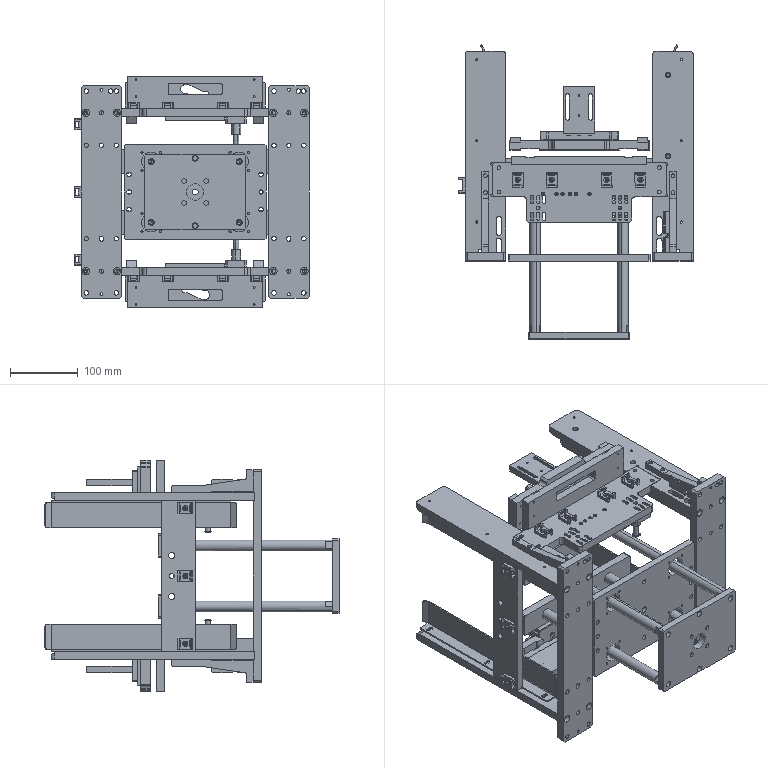Assembly | SolidWorks | mm | 65 component files | 65 solids | 2929 faces | box 346.2 x 434.2 x 342 mm | volume 3402690 mm3 | cylinder 1365 | plane 1260 | cone 216 | sphere 88 | commonest cylinder face diameters 0.6 x176 3.3 x164 4.5 x134 5.5 x96 6.6 x80 6 x79 4 x76 5 x66
Bill of materials:
01-1111 | 2 |  | Long, narrow, flat rectangular plate with small chamfered corners and an arrangement of round through holes laid out in rows, mostly three across, grouped near both ends and at about one-third and two-thirds of the length. Two small notches cut into one long edge.
02-1111 | 2 |  | Flat plate shaped like a T in plan. The wide main body has thinner, stepped-down tabs at each end, and each tab carries two round holes near its corners. A tab sticks out from one long edge, and near each of its ends sits a group of six parallel elongated slots arranged around a small central round hole.
03-1111 | 2 |  | Long rectangular bar with rounded corners at one end and a chamfered or angled edge at the same end. Near the other end it has a notched and stepped profile, a row of small holes, two elongated slots, and a hole in the end face. A long, shallow rectangular pocket or step is cut into one side edge in the middle of the bar, and there are a few widely spaced small holes on the top face.
04-1111 | 2 |  | Long rectangular bar very similar to unnamed part. It has the same stepped and notched end with an end-face hole, two slots and a small-hole cluster. It differs in having extra larger holes on the top face, a chamfer along the top edge at the far end, and a shallow step on the side edge where the other part has a long pocket.
05-1111 | 4 |  | Solid arm shaped roughly like an L. A tall rectangular block at one end has a horizontal round through hole. A tapered arm runs from the block, with its top surface sloping down to a level section near the far end. The level section has two vertical through holes, and there is a small step on the underside.
06-1111 | 4 |  | Long L-shaped angle that looks like bent sheet metal. It has an upright flange with rounded or chamfered end corners and a base flange with three elongated slots spaced along its length.
07-1111 | 1 |  | Rectangular bar or plate with four countersunk or conically shaped holes in one large face. Three round holes run along one narrow edge face, two larger and one smaller between them. There is a small step or rabbet along one long edge.
08-1111 | 2 |  | Thick, nearly square block with chamfered vertical corners. It has six round holes in two rows of three, with the middle hole of each row larger. A central hole has a larger counterbore or recess on the top face.
09-1111 | 4 |  | Small L-shaped bracket that looks like bent sheet metal. One flange has one long elongated slot. The other flange has two round holes near its outer corners. The outer corners are rounded.
10-1111 | 1 |  | Long, straight prismatic bar whose cross-section is a rectangle with one large angled chamfer, giving a five-sided profile. It has no holes or other features.
11-1111 | 2 |  | Stepped cylindrical pin. A slender shaft has a groove near its chamfered tip. The shaft joins a larger-diameter body that has one flat on its side. A short, reduced-diameter, chamfered spigot sits at the opposite end.
13-1111 | 2 |  | Thick rectangular plate with a rounded-rectangle through window in its upper middle. Five round holes run in a line near the bottom edge. Small holes sit near the end edges, shallow notches are cut into the top edge, and there is a step along one edge.
14-Z1-1111 | 2 |  | Elongated flat plate with a taller central section, an S-shaped curved through-slot, a 2x2 pattern of small holes on each end pad, and stepped thickness along the long edges.
17-1111 | 2 |  | Rectangular plate with two countersunk through-holes, chamfered top corners, and a stepped (L-shaped) cross-section.
18-1111 | 2 |  | Rectangular block with two long parallel through-slots and two small holes on the top face, three holes in one side face, and two lengthwise rectangular grooves on the underside.
19-1111 | 2 |  | I-shaped (dog-bone) bar: a narrow central web with three round through-holes, joining wider end pads that each have two elongated slots.
20-1111 | 4 |  | Thin flat rectangular plate with two elongated through-slots along its length and chamfered corners.
25-1111 | 4 |  | Rectangular bar with two round through-holes and a single angled bevel across one end.
21-1111 | 1 | S45C | Flat rectangular plate with four large circular openings, each surrounded by four small holes, plus medium holes on the centerline and along both short edges.
22-BF-1111 | 4 | 40CR | Long, slender cylindrical tube or rod with a central bore and a short, smaller-diameter step at one end.
23-1111 | 1 | A6061 | Flat rectangular plate with a large central through-bore, four small holes in a square around it, six perimeter holes, and chamfered corners.
24-1111 | 2 | A6061 | Flat rectangular bar with rounded corners and two counterbored through-holes near the ends.
RetainingRing~STWN8~MISUMI-1111 | 2 |  | Thin flat ring with a protruding tab that has an elongated slot; a split line passes radially through the tab and slot.
WireClip~M4-02~-1111 | 11 | PEEK | Rectangular block with a C/bracket-shaped profile: a solid base with a central round through-hole, and two raised end walls with inward lips forming rectangular through-passages.
Mates:
1. coincident | 01-1111-1 face at (-135.072, 406.224, 1393.056) dir (0, 1, 0) | 03-1111-1 face at (-135.072, 406.224, 1510.056) dir (0, -1, 0)
2. width | 01-1111-1 face at (-105.072, 408.224, 1236.056) dir (1, 0, 0) | 01-1111-1 face at (-165.072, 408.224, 1236.056) dir (-1, 0, 0) | 03-1111-1 face at (-165.072, 406.224, 1504.056) dir (-1, 0, 0) | 03-1111-1 face at (-105.072, 406.224, 1504.056) dir (1, 0, 0)
3. width | 03-1111-1 face at (-165.072, 406.224, 1516.056) dir (0, 0, 1) | 03-1111-1 face at (-165.072, 406.224, 1504.056) dir (0, 0, -1) | 01-1111-1 face at (-165.072, 406.224, 1516.056) dir (0, 0, -1) | 01-1111-1 face at (-165.072, 406.224, 1504.056) dir (0, 0, 1)
4. width | 04-1111-1 face at (-105.072, 406.224, 1270.056) dir (1, 0, 0) | 04-1111-1 face at (-165.072, 406.224, 1270.056) dir (-1, 0, 0) | 01-1111-1 face at (-105.072, 408.224, 1236.056) dir (1, 0, 0) | 01-1111-1 face at (-165.072, 408.224, 1236.056) dir (-1, 0, 0)
5. coincident | 01-1111-1 face at (-165.072, 408.224, 1550.056) dir (0, 0, 1) | 01-1111-2 face at (111.928, 408.224, 1550.056) dir (0, 0, 1)
6. coincident | 01-1111-1 face at (-135.072, 396.224, 1393.056) dir (0, -1, 0) | 01-1111-2 face at (141.928, 396.224, 1393.056) dir (0, -1, 0)
7. coincident | 01-1111-1 face at (-135.072, 408.224, 1393.056) dir (0, 1, 0) | 05-1111-1 face at (-140.072, 408.224, 1516.056) dir (0, -1, 0)
8. width | 01-1111-1 face at (-105.072, 408.224, 1236.056) dir (1, 0, 0) | 01-1111-1 face at (-165.072, 408.224, 1236.056) dir (-1, 0, 0) | 05-1111-1 face at (-140.072, 468.224, 1533.056) dir (-1, 0, 0) | 05-1111-1 face at (-130.072, 468.224, 1533.056) dir (1, 0, 0)
9. coincident | 01-1111-1 face at (-135.072, 408.224, 1393.056) dir (0, 1, 0) | 05-1111-3 face at (-130.072, 408.224, 1270.056) dir (0, -1, 0)
10. width | 01-1111-1 face at (-105.072, 408.224, 1236.056) dir (1, 0, 0) | 01-1111-1 face at (-165.072, 408.224, 1236.056) dir (-1, 0, 0) | 05-1111-3 face at (-140.072, 468.224, 1253.056) dir (-1, 0, 0) | 05-1111-3 face at (-130.072, 468.224, 1253.056) dir (1, 0, 0)
11. coincident | 03-1111-1 face at (-165.072, 406.224, 1516.056) dir (0, 0, 1) | 05-1111-1 face at (-140.072, 528.224, 1516.056) dir (0, 0, -1)
12. width | 03-1111-1 face at (-165.072, 406.224, 1516.056) dir (0, 0, 1) | 04-1111-1 face at (-165.072, 406.224, 1270.056) dir (0, 0, -1) | 07-1111-1 face at (-153.072, 543.224, 1282.056) dir (0, 0, -1) | 07-1111-1 face at (-153.072, 543.224, 1504.056) dir (0, 0, 1)
13. coincident | 04-1111-1 face at (-135.072, 706.224, 1276.056) dir (0, 0, -1) | 02-1111-3 face at (3.428, 516.224, 1276.056) dir (0, 0, 1)
14. width | 04-1111-1 face at (-105.072, 541.224, 1276.056) dir (0, -1, 0) | 04-1111-1 face at (-105.072, 491.224, 1276.056) dir (0, 1, 0) | 02-1111-3 face at (131.928, 491.224, 1282.056) dir (0, -1, 0) | 02-1111-3 face at (131.928, 541.224, 1282.056) dir (0, 1, 0)
15. coincident | 04-1111-1 face at (-105.072, 406.224, 1270.056) dir (1, 0, 0) | 02-1111-3 face at (-105.072, 491.224, 1276.056) dir (-1, 0, 0)
16. coincident | 04-1111-1 face at (-165.072, 406.224, 1270.056) dir (0, 0, -1) | 05-1111-3 face at (-130.072, 528.224, 1270.056) dir (0, 0, 1)
17. coincident | 04-1111-1 face at (-165.072, 406.224, 1282.056) dir (0, 0, 1) | 06-1111-6 face at (-135.572, 441.224, 1282.056) dir (0, 0, -1)
18. coincident | 04-1111-1 face at (-135.072, 706.224, 1276.056) dir (0, 1, 0) | 06-1111-6 face at (-138.308, 706.224, 1284.792) dir (0, 1, 0)
19. distance | 06-1111-6 face at (-135.572, 441.224, 1322.056) dir (1, 0, 0) | 04-1111-1 face at (-105.072, 406.224, 1270.056) dir (1, 0, 0)
20. width | 04-1111-2 face at (171.928, 406.224, 1516.056) dir (0, 0, 1) | 04-1111-2 face at (171.928, 406.224, 1504.056) dir (0, 0, -1) | 01-1111-2 face at (111.928, 406.224, 1504.056) dir (0, 0, 1) | 01-1111-2 face at (111.928, 406.224, 1516.056) dir (0, 0, -1)
21. width | 04-1111-2 face at (171.928, 406.224, 1516.056) dir (1, 0, 0) | 04-1111-2 face at (111.928, 406.224, 1516.056) dir (-1, 0, 0) | 01-1111-2 face at (171.928, 408.224, 1236.056) dir (1, 0, 0) | 01-1111-2 face at (111.928, 408.224, 1236.056) dir (-1, 0, 0)
22. width | 01-1111-2 face at (111.928, 406.224, 1282.056) dir (0, 0, -1) | 01-1111-2 face at (111.928, 406.224, 1270.056) dir (0, 0, 1) | 03-1111-2 face at (171.928, 406.224, 1270.056) dir (0, 0, -1) | 03-1111-2 face at (171.928, 406.224, 1282.056) dir (0, 0, 1)
23. width | 03-1111-2 face at (111.928, 406.224, 1282.056) dir (-1, 0, 0) | 03-1111-2 face at (171.928, 406.224, 1282.056) dir (1, 0, 0) | 01-1111-2 face at (171.928, 408.224, 1236.056) dir (1, 0, 0) | 01-1111-2 face at (111.928, 408.224, 1236.056) dir (-1, 0, 0)
24. coincident | 01-1111-2 face at (141.928, 408.224, 1393.056) dir (0, 1, 0) | 05-1111-2 face at (136.928, 408.224, 1516.056) dir (0, -1, 0)
25. width | 01-1111-2 face at (111.928, 408.224, 1236.056) dir (-1, 0, 0) | 01-1111-2 face at (171.928, 408.224, 1236.056) dir (1, 0, 0) | 05-1111-2 face at (136.928, 468.224, 1533.056) dir (-1, 0, 0) | 05-1111-2 face at (146.928, 468.224, 1533.056) dir (1, 0, 0)
26. coincident | 01-1111-2 face at (141.928, 408.224, 1393.056) dir (0, 1, 0) | 05-1111-4 face at (146.928, 408.224, 1270.056) dir (0, -1, 0)
27. width | 01-1111-2 face at (111.928, 408.224, 1236.056) dir (-1, 0, 0) | 01-1111-2 face at (171.928, 408.224, 1236.056) dir (1, 0, 0) | 05-1111-4 face at (146.928, 468.224, 1253.056) dir (1, 0, 0) | 05-1111-4 face at (136.928, 468.224, 1253.056) dir (-1, 0, 0)
28. coincident | 03-1111-2 face at (171.928, 406.224, 1270.056) dir (0, 0, -1) | 05-1111-4 face at (146.928, 528.224, 1270.056) dir (0, 0, 1)
29. coincident | 04-1111-2 face at (171.928, 406.224, 1516.056) dir (0, 0, 1) | 05-1111-2 face at (136.928, 528.224, 1516.056) dir (0, 0, -1)
30. coincident | 04-1111-2 face at (171.928, 406.224, 1504.056) dir (0, 0, -1) | 06-1111-5 face at (142.428, 441.224, 1504.056) dir (0, 0, 1)
31. coincident | 04-1111-2 face at (141.928, 706.224, 1510.056) dir (0, 1, 0) | 06-1111-5 face at (145.165, 706.224, 1501.319) dir (0, 1, 0)
32. distance | 06-1111-5 face at (142.428, 441.224, 1464.056) dir (-1, 0, 0) | 04-1111-2 face at (111.928, 406.224, 1516.056) dir (-1, 0, 0)
33. coincident | 04-1111-1 face at (-165.072, 406.224, 1270.056) dir (-1, 0, 0) | 07-1111-1 face at (-165.072, 518.224, 1393.056) dir (-1, 0, 0)
34. coincident | 04-1111-2 face at (171.928, 406.224, 1516.056) dir (0, 0, 1) | 09-1111-1 face at (147.928, 399.224, 1516.056) dir (0, 0, -1)
35. parallel | 04-1111-2 face at (141.928, 706.224, 1510.056) dir (0, 1, 0) | 09-1111-1 face at (129.928, 431.224, 1518.792) dir (0, 1, 0)
36. distance | 09-1111-1 face at (147.928, 399.224, 1518.056) dir (1, 0, 0) | 04-1111-2 face at (171.928, 406.224, 1516.056) dir (1, 0, 0)
37. distance | 09-1111-1 face at (129.928, 431.224, 1518.792) dir (0, 1, 0) | 04-1111-2 face at (141.928, 706.224, 1510.056) dir (0, 1, 0)
38. coincident | 09-1111-1 face at (129.928, 431.224, 1518.792) dir (0, 1, 0) | 09-1111-12 face at (130.665, 431.224, 1267.319) dir (0, 1, 0)
39. coincident | 09-1111-1 face at (127.928, 399.224, 1516.056) dir (-1, 0, 0) | 09-1111-12 face at (127.928, 431.224, 1270.056) dir (-1, 0, 0)
40. coincident | 03-1111-2 face at (171.928, 406.224, 1270.056) dir (0, 0, -1) | 09-1111-12 face at (147.928, 431.224, 1270.056) dir (0, 0, 1)
41. coincident | 04-1111-1 face at (-165.072, 406.224, 1282.056) dir (0, 0, 1) | 10-1111-1 face at (-135.572, 406.224, 1282.056) dir (0, 0, -1)
42. coincident | 06-1111-6 face at (-135.572, 441.224, 1322.056) dir (1, 0, 0) | 10-1111-1 face at (-135.572, 406.224, 1282.056) dir (-1, 0, 0)
43. distance | 10-1111-1 face at (-128.072, 696.224, 1291.056) dir (0, 1, 0) | 04-1111-1 face at (-135.072, 706.224, 1276.056) dir (0, 1, 0)
44. distance | 07-1111-1 face at (-153.072, 543.224, 1282.056) dir (0, 1, 0) | 01-1111-1 face at (-135.072, 408.224, 1393.056) dir (0, 1, 0)
45. coincident | 11-1111-1 face at (63.928, 474.724, 1327.156) dir (0, 0, 1) | RetainingRing~STWN8~MISUMI-1111-1 face at (70.259, 473.944, 1327.156) dir (0, 0, -1)
46. concentric | 11-1111-1 face at (63.928, 474.724, 1290.056) dir (0, 0, -1) r 4 | RetainingRing~STWN8~MISUMI-1111-1 face at (63.928, 474.724, 1327.956) dir (0, 0, 1) r 3.8
47. coincident | 03-1111-1 face at (-135.072, 706.224, 1510.056) dir (0, 0, 1) | 02-1111-4 face at (3.428, 516.224, 1510.056) dir (0, 0, -1)
48. width | 02-1111-4 face at (-125.072, 541.224, 1504.056) dir (0, 1, 0) | 02-1111-4 face at (-125.072, 491.224, 1504.056) dir (0, -1, 0) | 03-1111-1 face at (-105.072, 541.224, 1510.056) dir (0, -1, 0) | 03-1111-1 face at (-105.072, 491.224, 1510.056) dir (0, 1, 0)
49. coincident | 03-1111-1 face at (-125.072, 541.224, 1510.056) dir (1, 0, 0) | 02-1111-4 face at (-125.072, 541.224, 1504.056) dir (-1, 0, 0)
50. coincident | 04-1111-2 face at (131.928, 541.224, 1510.056) dir (-1, 0, 0) | 02-1111-4 face at (131.928, 541.224, 1504.056) dir (1, 0, 0)
51. profile center | 11-1111-1 face at (64.268, 479.713, 1290.056) dir (0, 0, -1) | 08-1111-2 face at (63.928, 474.724, 1290.056) dir (0, 0, 1)
52. profile center | 11-1111-2 face at (60.777, 478.607, 1496.056) dir (0, 0, 1) | 08-1111-3 face at (63.928, 474.724, 1496.056) dir (0, 0, -1)
53. concentric | 11-1111-2 face at (63.928, 474.724, 1496.056) dir (0, 0, 1) r 4 | RetainingRing~STWN8~MISUMI-1111-2 face at (63.928, 474.724, 1458.956) dir (0, 0, 1) r 3.8
54. coincident | 11-1111-2 face at (63.928, 474.724, 1458.956) dir (0, 0, -1) | RetainingRing~STWN8~MISUMI-1111-2 face at (70.258, 473.937, 1458.956) dir (0, 0, 1)
55. coincident | 02-1111-4 face at (3.428, 516.224, 1504.056) dir (0, 0, -1) | 08-1111-3 face at (63.928, 474.724, 1504.056) dir (0, 0, 1)
56. concentric | 02-1111-4 face at (63.928, 474.724, 1504.056) dir (0, 0, 1) r 2.75 | 08-1111-3 face at (63.928, 474.724, 1504.056) dir (0, 0, 1) r 5
57. parallel | 02-1111-4 face at (80.928, 453.224, 1516.056) dir (1, 0, 0) | 08-1111-3 face at (78.928, 492.224, 1504.056) dir (1, 0, 0)
58. concentric | 02-1111-3 face at (63.928, 474.724, 1282.056) dir (0, 0, -1) r 2.75 | 08-1111-2 face at (63.928, 474.724, 1282.056) dir (0, 0, -1) r 5
59. coincident | 02-1111-3 face at (3.428, 516.224, 1282.056) dir (0, 0, 1) | 08-1111-2 face at (63.928, 474.724, 1282.056) dir (0, 0, -1)
60. parallel | 02-1111-3 face at (80.928, 453.224, 1270.056) dir (1, 0, 0) | 08-1111-2 face at (78.928, 492.224, 1282.056) dir (1, 0, 0)
61. coincident | 03-1111-2 face at (171.928, 406.224, 1282.056) dir (0, 0, 1) | 06-1111-3 face at (142.428, 706.224, 1282.056) dir (0, 0, -1)
62. distance | 06-1111-3 face at (142.428, 706.224, 1322.056) dir (-1, 0, 0) | 03-1111-2 face at (111.928, 406.224, 1282.056) dir (-1, 0, 0)
63. coincident | 03-1111-2 face at (141.928, 706.224, 1276.056) dir (0, 1, 0) | 06-1111-3 face at (144.428, 706.224, 1284.792) dir (0, 1, 0)
64. coincident | 03-1111-1 face at (-165.072, 406.224, 1504.056) dir (0, 0, -1) | 06-1111-4 face at (-135.572, 706.224, 1504.056) dir (0, 0, 1)
65. distance | 06-1111-4 face at (-135.572, 706.224, 1464.056) dir (1, 0, 0) | 03-1111-1 face at (-105.072, 406.224, 1504.056) dir (1, 0, 0)
66. coincident | 03-1111-1 face at (-135.072, 706.224, 1510.056) dir (0, 1, 0) | 06-1111-4 face at (-137.572, 706.224, 1501.319) dir (0, 1, 0)
67. coincident | 02-1111-3 face at (3.428, 516.224, 1270.056) dir (0, 0, -1) | 12-DividingMechanism-1111-2/13-1111-1 face at (103.428, 541.224, 1270.056) dir (0, 0, 1)
68. coincident | 02-1111-3 face at (131.928, 541.224, 1282.056) dir (0, 1, 0) | 12-DividingMechanism-1111-2/13-1111-1 face at (3.428, 541.224, 1252.056) dir (0, -1, 0)
69. coincident | 02-1111-4 face at (-125.072, 541.224, 1504.056) dir (0, 1, 0) | 12-DividingMechanism-1111-1/13-1111-1 face at (3.428, 541.224, 1534.056) dir (0, -1, 0)
70. coincident | 02-1111-4 face at (3.428, 516.224, 1516.056) dir (0, 0, 1) | 12-DividingMechanism-1111-1/13-1111-1 face at (-96.572, 541.224, 1516.056) dir (0, 0, -1)
71. coincident | 01-1111-1 face at (-135.072, 396.224, 1393.056) dir (0, -1, 0) | 20-MaterialTrayLifting-1111-1/21-1111-1 face at (3.428, 396.224, 1393.056) dir (0, -1, 0)
72. width | 01-1111-1 face at (-165.072, 408.224, 1236.056) dir (0, 0, -1) | 01-1111-1 face at (-165.072, 408.224, 1550.056) dir (0, 0, 1) | 20-MaterialTrayLifting-1111-1/21-1111-1 face at (-101.572, 406.224, 1323.056) dir (0, 0, -1) | 20-MaterialTrayLifting-1111-1/21-1111-1 face at (-101.572, 406.224, 1463.056) dir (0, 0, 1)
73. width | 01-1111-1 face at (-105.072, 408.224, 1236.056) dir (1, 0, 0) | 01-1111-2 face at (111.928, 408.224, 1236.056) dir (-1, 0, 0) | 20-MaterialTrayLifting-1111-1/21-1111-1 face at (-101.572, 406.224, 1323.056) dir (-1, 0, 0) | 20-MaterialTrayLifting-1111-1/21-1111-1 face at (108.428, 406.224, 1323.056) dir (1, 0, 0)
74. concentric | 02-1111-4 face at (93.928, 516.224, 1516.056) dir (0, 0, 1) r 1.65 | WireClip~M4-02~-1111-3 face at (93.928, 516.224, 1520.356) dir (0, 0, 1) r 2.25
75. coincident | WireClip~M4-02~-1111-5 face at (-45.005, 507.861, 1520.356) dir (0, 0, 1) | WireClip~M4-02~-1111-6 face at (-95.005, 507.861, 1520.356) dir (0, 0, 1)
76. coincident | WireClip~M4-02~-1111-4 face at (35.995, 507.861, 1520.356) dir (0, 0, 1) | WireClip~M4-02~-1111-5 face at (-45.005, 507.861, 1520.356) dir (0, 0, 1)
77. coincident | WireClip~M4-02~-1111-3 face at (85.995, 507.861, 1520.356) dir (0, 0, 1) | WireClip~M4-02~-1111-4 face at (35.995, 507.861, 1520.356) dir (0, 0, 1)
78. concentric | 02-1111-4 face at (43.928, 516.224, 1516.056) dir (0, 0, 1) r 1.65 | WireClip~M4-02~-1111-4 face at (43.928, 516.224, 1520.356) dir (0, 0, 1) r 4
79. concentric | 02-1111-4 face at (-37.072, 516.224, 1516.056) dir (0, 0, 1) r 1.65 | WireClip~M4-02~-1111-5 face at (-37.072, 516.224, 1520.356) dir (0, 0, 1) r 4
80. concentric | 02-1111-4 face at (-87.072, 516.224, 1516.056) dir (0, 0, 1) r 1.65 | WireClip~M4-02~-1111-6 face at (-87.072, 516.224, 1520.356) dir (0, 0, 1) r 4
81. coincident | 07-1111-1 face at (-165.072, 518.224, 1393.056) dir (-1, 0, 0) | WireClip~M4-02~-1111-11 face at (-165.072, 496.988, 1401.145) dir (1, 0, 0)
82. concentric | 07-1111-1 face at (-165.072, 508.224, 1393.056) dir (-1, 0, 0) r 1.65 | WireClip~M4-02~-1111-11 face at (-169.372, 508.224, 1393.056) dir (-1, 0, 0) r 4
83. coincident | WireClip~M4-02~-1111-14 face at (-169.372, 499.861, 1285.122) dir (-1, 0, 0) | WireClip~M4-02~-1111-15 face at (-169.372, 499.861, 1485.122) dir (-1, 0, 0)
84. coincident | WireClip~M4-02~-1111-11 face at (-169.372, 499.861, 1385.122) dir (-1, 0, 0) | WireClip~M4-02~-1111-14 face at (-169.372, 499.861, 1285.122) dir (-1, 0, 0)
85. concentric | 07-1111-1 face at (-165.072, 508.224, 1493.056) dir (-1, 0, 0) r 1.65 | WireClip~M4-02~-1111-15 face at (-169.372, 508.224, 1493.056) dir (-1, 0, 0) r 4
86. concentric | 07-1111-1 face at (-165.072, 508.224, 1293.056) dir (-1, 0, 0) r 1.65 | WireClip~M4-02~-1111-14 face at (-169.372, 508.224, 1293.056) dir (-1, 0, 0) r 4
87. coincident | 04-1111-1 face at (-165.072, 406.224, 1282.056) dir (0, 0, 1) | 07-1111-1 face at (-153.072, 543.224, 1282.056) dir (0, 0, -1)
88. width | 01-1111-1 face at (-165.072, 408.224, 1236.056) dir (0, 0, -1) | 01-1111-1 face at (-165.072, 408.224, 1550.056) dir (0, 0, 1) | 04-1111-1 face at (-165.072, 406.224, 1270.056) dir (0, 0, -1) | 03-1111-1 face at (-165.072, 406.224, 1516.056) dir (0, 0, 1)
89. coincident | 03-1111-1 face at (-165.072, 406.224, 1516.056) dir (0, 0, 1) | 04-1111-2 face at (171.928, 406.224, 1516.056) dir (0, 0, 1)
90. coincident | 03-1111-2 face at (171.928, 406.224, 1270.056) dir (0, 0, -1) | 04-1111-1 face at (-165.072, 406.224, 1270.056) dir (0, 0, -1)
91. coincident | 01-1111-1 face at (-135.072, 396.224, 1393.056) dir (0, -1, 0) | 01-1111-2 face at (141.928, 396.224, 1393.056) dir (0, -1, 0)
92. width | 03-1111-2 face at (111.928, 406.224, 1282.056) dir (-1, 0, 0) | 04-1111-1 face at (-105.072, 406.224, 1270.056) dir (1, 0, 0) | 12-DividingMechanism-1111-2/14-Z1-1111-1 face at (106.678, 573.824, 1222.056) dir (1, 0, 0) | 12-DividingMechanism-1111-2/14-Z1-1111-1 face at (-99.822, 573.824, 1222.056) dir (-1, 0, 0)
93. coincident | 12-DividingMechanism-1111-1/14-Z1-1111-1 face at (-99.822, 573.824, 1564.056) dir (-1, 0, 0) | 12-DividingMechanism-1111-2/14-Z1-1111-1 face at (-99.822, 573.824, 1222.056) dir (-1, 0, 0)
94. coincident | 01-1111-1 face at (-135.072, 406.224, 1393.056) dir (0, 1, 0) | 04-1111-1 face at (-135.072, 406.224, 1276.056) dir (0, -1, 0)
95. coincident | 01-1111-2 face at (141.928, 406.224, 1393.056) dir (0, 1, 0) | 04-1111-2 face at (141.928, 406.224, 1510.056) dir (0, -1, 0)
96. coincident | 01-1111-2 face at (141.928, 406.224, 1393.056) dir (0, 1, 0) | 03-1111-2 face at (141.928, 406.224, 1276.056) dir (0, -1, 0)
97. coincident | WireClip~M4-02~-1111-3 face at (102.018, 504.988, 1516.056) dir (0, 0, -1) | 02-1111-4 face at (3.428, 516.224, 1516.056) dir (0, 0, 1)
98. width | 14-Z1-1111-1 face at (-53.322, 600.824, 1587.056) dir (-1, 0, 0) | 14-Z1-1111-1 face at (153.178, 600.824, 1587.056) dir (1, 0, 0) | 13-1111-1 face at (149.928, 578.224, 1587.056) dir (1, 0, 0) | 13-1111-1 face at (-50.072, 578.224, 1587.056) dir (-1, 0, 0)
99. coincident | 14-Z1-1111-1 face at (49.928, 598.824, 1557.056) dir (0, 1, 0) | 25-1111-2 face at (-43.822, 598.824, 1547.056) dir (0, -1, 0)
100. width | 14-Z1-1111-1 face at (-36.322, 598.824, 1527.056) dir (-1, 0, 0) | 14-Z1-1111-1 face at (-51.322, 598.824, 1527.056) dir (1, 0, 0) | 25-1111-2 face at (-51.322, 606.024, 1517.056) dir (-1, 0, 0) | 25-1111-2 face at (-36.322, 606.024, 1517.056) dir (1, 0, 0)
101. coincident | 14-Z1-1111-1 face at (-53.322, 587.224, 1577.056) dir (0, 0, 1) | 25-1111-2 face at (-36.322, 606.024, 1577.056) dir (0, 0, 1)
102. coincident | 14-Z1-1111-1 face at (49.928, 598.824, 1557.056) dir (0, 1, 0) | 25-1111-3 face at (143.678, 598.824, 1547.056) dir (0, -1, 0)
103. width | 25-1111-3 face at (136.178, 606.024, 1517.056) dir (-1, 0, 0) | 25-1111-3 face at (151.178, 606.024, 1517.056) dir (1, 0, 0) | 14-Z1-1111-1 face at (136.178, 598.824, 1527.056) dir (1, 0, 0) | 14-Z1-1111-1 face at (151.178, 598.824, 1527.056) dir (-1, 0, 0)
104. coincident | 14-Z1-1111-1 face at (153.178, 587.224, 1577.056) dir (0, 0, 1) | 25-1111-3 face at (151.178, 606.024, 1577.056) dir (0, 0, 1)
105. coincident | 18-1111-3 face at (26.928, 611.924, 1559.056) dir (0, -1, 0) | 19-1111-5 face at (49.928, 611.924, 1554.056) dir (0, 1, 0)
106. width | 19-1111-5 face at (-7.572, 613.924, 1536.556) dir (-1, 0, 0) | 19-1111-5 face at (107.428, 613.924, 1536.556) dir (1, 0, 0) | 18-1111-3 face at (72.928, 611.924, 1559.056) dir (1, 0, 0) | 18-1111-3 face at (26.928, 611.924, 1559.056) dir (-1, 0, 0)
107. coincident | 18-1111-3 face at (49.928, 646.474, 1559.056) dir (0, 0, 1) | 19-1111-5 face at (2.428, 602.924, 1559.056) dir (0, 0, 1)
108. width | 14-Z1-1111-1 face at (153.178, 600.824, 1587.056) dir (1, 0, 0) | 14-Z1-1111-1 face at (-53.322, 600.824, 1587.056) dir (-1, 0, 0) | 19-1111-5 face at (-7.572, 613.924, 1536.556) dir (-1, 0, 0) | 19-1111-5 face at (107.428, 613.924, 1536.556) dir (1, 0, 0)
109. distance | 14-Z1-1111-1 face at (-53.322, 600.824, 1527.056) dir (0, 0, -1) | 13-1111-1 face at (-50.072, 578.224, 1527.056) dir (0, 0, -1)
110. coincident | 14-Z1-1111-1 face at (97.428, 587.224, 1549.056) dir (0, 0, -1) | 19-1111-5 face at (2.428, 602.924, 1549.056) dir (0, 0, -1)
111. coincident | 14-Z1-1111-1 face at (49.928, 600.824, 1557.056) dir (0, 1, 0) | 20-1111-3 face at (49.928, 600.824, 1554.056) dir (0, -1, 0)
112. coincident | 19-1111-5 face at (49.928, 602.924, 1554.056) dir (0, -1, 0) | 20-1111-3 face at (49.928, 602.924, 1554.056) dir (0, 1, 0)
113. concentric | 19-1111-5 face at (102.428, 613.924, 1541.306) dir (0, 1, 0) r 2.75 | 20-1111-3 face at (102.428, 602.924, 1541.306) dir (0, 1, 0) r 2.75
114. coincident | 19-1111-5 face at (49.928, 602.924, 1554.056) dir (0, -1, 0) | 20-1111-4 face at (-55.072, 602.924, 1554.056) dir (0, 1, 0)
115. concentric | 19-1111-5 face at (-2.572, 613.924, 1562.306) dir (0, 1, 0) r 2.75 | 20-1111-4 face at (-2.572, 602.924, 1562.306) dir (0, 1, 0) r 2.75
116. profile center | 24-1111-3 face at (258.464, 105.27, 226.33) dir (0, -1, 0) | 22-BF-1111-11 face at (258.464, 105.27, 226.33) dir (0, 1, 0)
117. profile center | 22-BF-1111-12 face at (128.464, 105.27, 226.33) dir (0, 1, 0) | 24-1111-3 face at (128.464, 105.27, 226.33) dir (0, -1, 0)
118. profile center | 24-1111-4 face at (128.464, 105.27, 116.33) dir (0, -1, 0) | 22-BF-1111-10 face at (128.464, 105.27, 116.33) dir (0, 1, 0)
119. profile center | 22-BF-1111-9 face at (258.464, 105.27, 116.33) dir (0, 1, 0) | 24-1111-4 face at (258.464, 105.27, 116.33) dir (0, -1, 0)
120. coincident | 24-1111-3 face at (83.464, 114.27, 243.83) dir (0, 1, 0) | 24-1111-4 face at (83.464, 114.27, 133.83) dir (0, 1, 0)
121. coincident | 22-BF-1111-9 face at (258.464, -144.73, 116.33) dir (0, -1, 0) | 23-1111-2 face at (258.464, -144.73, 116.33) dir (0, 1, 0)
122. parallel | 21-1111-1 face at (88.464, -27.73, 91.33) dir (0, 0, -1) | 23-1111-2 face at (118.464, -152.73, 106.33) dir (0, 0, -1)
123. concentric | 22-BF-1111-9 face at (258.464, -144.73, 116.33) dir (0, 1, 0) r 8 | 23-1111-2 face at (258.464, -152.73, 116.33) dir (0, -1, 0) r 4.5
124. distance | 23-1111-2 face at (193.464, -142.73, 161.33) dir (0, 1, 0) | 21-1111-1 face at (193.464, -37.73, 161.33) dir (0, -1, 0)